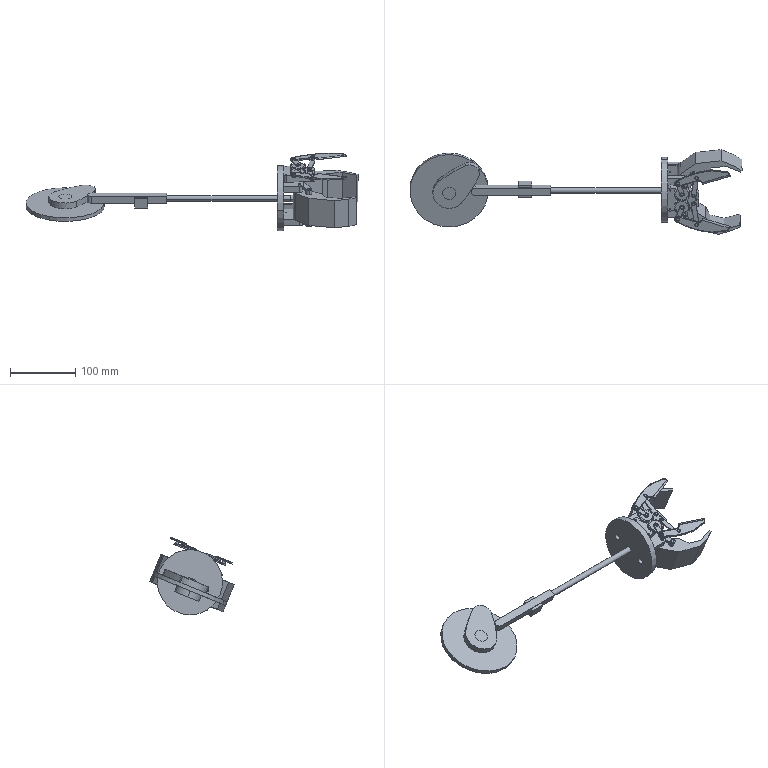Assembly | SolidWorks | mm | 30 component files | 31 solids | 649 faces | box 508.98 x 129.73 x 119.11 mm | volume 396416 mm3 | cylinder 341 | plane 286 | cone 16 | torus 4 | sphere 2 | commonest cylinder face diameters 4 x54 0.6 x54 5 x40 24 x40 5.6 x20 2.2 x14 8.636 x14 10 x12
Bill of materials:
2026.08.03FixedRail | 1 |  | Rectangular prismatic block with a rectangular slot running its full length, so its constant cross-section is a U-channel.
2026.08.03NewSchemeConnectingRod | 1 |  | Long straight bar with a square cross-section. One end is rounded. The other end face has a centered round blind hole whose bottom looks conical.
Cam | 1 |  | Flat plate of uniform thickness with a teardrop or cam-like outline. It has a single round through-hole near the center of the larger rounded end.
ConnectingRod | 2 |  | Flat straight link with an obround outline. It has two round through-holes, one at the center of each rounded end, and constant thickness.
ConnectingRod-B | 1 |  | Straight link with two through-holes. One end carries a taller cylindrical boss that sticks out from one face only, which gives an L-shaped side profile.
EccentricWheel | 1 |  | Thin circular disc with a small cylindrical pin or boss at its center. The pin appears to stick out from both faces.
FixedBushing | 1 |  | Plain thick ring with a rectangular cross-section: a cylindrical outer surface and a concentric cylindrical bore.
Holding Part | 1 |  | Thick plate with a trapezoidal outline and rounded corners. It has seven round through-holes: two small holes near the wide end, four larger holes in a roughly rectangular pattern, and one small hole near the narrow end.
Long Arm | 1 |  | Flat straight link with an obround outline and constant thickness. It has two round through-holes, one at the center of each rounded end.
MirrorConnectingRod-B | 1 |  | Straight link with two through-holes. A taller cylindrical boss at one end extends from one face, which gives an L-shaped side profile.
MirrorLong Arm | 1 |  | Flat straight link with an obround outline and constant thickness. It has two round through-holes, one at each rounded end.
Mirrorpin | 1 |  | Solid cylinder with a rectangular key or rib running lengthwise along one side. The key covers only part of the cylinder's length, starting at or near one end.
Mirrorpin2 | 3 |  | Plain solid right circular cylinder with flat ends.
MirrorShort Arm | 1 |  | Flat link plate (bar with rounded ends) with a through hole at each end; one hole has a small rectangular keyway notch.
MirrorSimple Gear | 1 |  | Flat spur-gear-like disc with straight-sided, roughly trapezoidal teeth and a central bore with keyway-type notches.
MirrorThe Claw | 1 |  | Thin flat blade-shaped plate with two small holes in a narrow shank and a wider tapering blade section with a bevelled edge.
Part1(1) | 1 |  | Circular flange disc with two parallel rectangular plate brackets sticking out from one face; the brackets and disc have several holes.
pin | 1 |  | Solid cylinder with a rectangular key-like rib running along the full length of its side.
pin2 | 3 |  | Plain solid right circular cylinder with flat ends.
RightJaw | 2 |  | Thick bracket or lever with a bent profile: one rounded end with a through hole, a small cylindrical pin sticking out of both faces, and an angled arm.
Short Arm | 1 |  | Flat link plate with rounded ends and two end holes; one hole has a small keyway notch.
Simple Gear | 1 |  | Flat spur-gear-like disc with straight-sided teeth and a central bore with keyway-type notches.
TelescopicRod | 1 |  | Long thin round rod ending in a short perpendicular cross-bar, forming a T, with a ball-shaped node where they meet.
The Claw | 1 |  | Thin flat blade-shaped plate with two holes in a narrow shank and a wider section with a bevelled long edge and an angled tip.
Mates:
1. concentric | Part1(1)-1 face at (323.621, 37.527, 8.706) dir (0, 0.3818, -0.9242) r 2.5 | RightJaw-1 face at (323.621, 20.343, 50.296) dir (0, 0.3818, -0.9242) r 2.5
2. coincident | Part1(1)-1 face at (328.621, 42.148, 10.615) dir (0, -0.3818, 0.9242) | RightJaw-2 face at (323.621, -13.306, -12.296) dir (0, 0.3818, -0.9242)
3. concentric | Part1(1)-1 face at (323.621, -13.306, -12.296) dir (0, 0.3818, -0.9242) r 2.5 | RightJaw-2 face at (323.621, -13.306, -12.296) dir (0, -0.3818, 0.9242) r 2.5
4. concentric | RightJaw-1 face at (338.214, 48.015, 4.383) dir (0, -0.3818, 0.9242) r 2.5 | ConnectingRod-1 face at (338.214, 46.488, 8.08) dir (0, -0.3818, 0.9242) r 2.5
5. coincident | RightJaw-1 face at (323.621, 37.527, 8.706) dir (0, 0.3818, -0.9242) | ConnectingRod-1 face at (338.214, 44.961, 11.777) dir (0, -0.3818, 0.9242)
6. concentric | RightJaw-2 face at (337.105, -19.3, -23.428) dir (0, -0.3818, 0.9242) r 2.5 | ConnectingRod-B-1 face at (337.105, -20.827, -19.731) dir (0, 0.3818, -0.9242) r 2.5
7. concentric | TelescopicRod-1 face at (321.124, -8.702, 46.952) dir (0, 0.3818, -0.9242) r 2.5 | ConnectingRod-1 face at (321.124, 13.063, -5.729) dir (0, -0.3818, 0.9242) r 2.5
8. concentric | TelescopicRod-1 face at (321.124, -8.702, 46.952) dir (0, 0.3818, -0.9242) r 2.5 | ConnectingRod-B-1 face at (321.124, 13.063, -5.729) dir (0, 0.3818, -0.9242) r 2.5
9. coincident | ConnectingRod-1 face at (338.214, 46.488, 8.08) dir (0, 0.3818, -0.9242) | ConnectingRod-B-1 face at (321.124, 13.063, -5.729) dir (0, -0.3818, 0.9242)
10. coincident | ConnectingRod-2 face at (338.214, 26.25, 57.064) dir (0, -0.3818, 0.9242) | MirrorConnectingRod-B-2 face at (321.124, -7.175, 43.255) dir (0, 0.3818, -0.9242)
11. parallel | 2026.08.03FixedRail-1 face at (90.094, 11.482, 13.811) dir (0, -0.3818, 0.9242) | 2026.08.03NewSchemeConnectingRod-2 face at (3.551, 0.6532, 24.308) dir (0, -0.3818, 0.9242)
12. parallel | Part1(1)-1 face at (328.621, -38.929, 36.627) dir (0, -0.3818, 0.9242) | FixedBushing-2 face at (-36.329, 4.513, 6.427) dir (0, -0.3818, 0.9242)
13. concentric | FixedBushing-2 face at (-36.329, 4.513, 6.427) dir (0, 0.3818, -0.9242) r 12.5 | EccentricWheel-2 face at (-36.329, 8.332, -2.815) dir (0, -0.3818, 0.9242) r 12.5
14. concentric | EccentricWheel-2 face at (-36.329, -1.596, 21.215) dir (0, 0.3818, -0.9242) r 10 | Cam-1 face at (-36.329, 2.222, 11.972) dir (0, -0.3818, 0.9242) r 10
15. coincident | EccentricWheel-2 face at (-36.329, 2.222, 11.972) dir (0, -0.3818, 0.9242) | Cam-1 face at (-93.023, 69.986, 39.969) dir (0, 0.3818, -0.9242)
16. coincident | FixedBushing-2 face at (-36.329, 4.513, 6.427) dir (0, -0.3818, 0.9242) | EccentricWheel-2 face at (-36.329, 4.513, 6.427) dir (0, 0.3818, -0.9242)
17. coincident | 2026.08.03NewSchemeConnectingRod-2 face at (3.551, 5.235, 13.217) dir (0, 0.3818, -0.9242) | EccentricWheel-2 face at (-36.329, 2.222, 11.972) dir (0, -0.3818, 0.9242)
18. cam | Cam-1 face at (-181.218, 104.23, 64.937) dir (0, 0.3818, -0.9242) r 209.672 | 2026.08.03NewSchemeConnectingRod-2 face at (3.551, 0.6532, 24.308) dir (0, 0.3818, -0.9242) r 6
19. coincident | 2026.08.03FixedRail-1 face at (90.094, 0.3913, 9.229) dir (0, 0.9242, 0.3818) | 2026.08.03NewSchemeConnectingRod-2 face at (3.551, -4.892, 22.017) dir (0, -0.9242, -0.3818)
20. concentric | Part1(1)-1 face at (302.621, -16.981, 34.875) dir (0, -0.3818, 0.9242) r 1.1 | Holding Part-1 face at (302.621, -25.381, 55.208) dir (0, 0.3818, -0.9242) r 1.1
21. coincident | Part1(1)-1 face at (302.621, 11.176, 46.508) dir (0, -0.3818, 0.9242) r 1.1 | Holding Part-1 edge at (302.621, 2.775, 66.841) dir (0, -0.3818, 0.9242) r 1.1
22. coincident | Part1(1)-1 face at (328.621, -38.929, 36.627) dir (0, -0.3818, 0.9242) | Holding Part-1 face at (342.621, 0.8389, 53.057) dir (0, 0.3818, -0.9242)
23. coincident | Holding Part-1 face at (320.621, -0.9517, 65.301) dir (0, 0.3818, -0.9242) r 2 | Simple Gear-1 edge at (320.621, -2.479, 68.998) dir (0, 0.3818, -0.9242) r 2
24. coincident | Holding Part-1 face at (342.621, -3.743, 64.148) dir (0, -0.3818, 0.9242) | Simple Gear-1 face at (320.621, -0.9517, 65.301) dir (0, 0.3818, -0.9242)
25. concentric | Short Arm-1 face at (320.621, -2.479, 68.998) dir (0, -0.3818, 0.9242) r 2 | Simple Gear-1 face at (320.621, -0.9517, 65.301) dir (0, -0.3818, 0.9242) r 2
26. coincident | Short Arm-1 face at (320.621, -2.479, 68.998) dir (0, 0.3818, -0.9242) | Simple Gear-1 face at (320.621, -2.479, 68.998) dir (0, -0.3818, 0.9242)
27. concentric | Short Arm-1 face at (314.445, 14.655, 76.077) dir (0, -0.3818, 0.9242) r 2 | The Claw-1 face at (314.445, 13.127, 79.774) dir (0, 0.3818, -0.9242) r 2
28. coincident | Short Arm-1 face at (320.621, -3.243, 70.847) dir (0, -0.3818, 0.9242) | The Claw-1 face at (315.971, 9.49, 76.108) dir (0, 0.3818, -0.9242)
29. concentric | Holding Part-1 face at (338.621, -4.649, 63.774) dir (0, 0.3818, -0.9242) r 2 | Long Arm-1 face at (338.621, -4.649, 63.774) dir (0, -0.3818, 0.9242) r 2
30. coincident | Holding Part-1 face at (342.621, -3.743, 64.148) dir (0, -0.3818, 0.9242) | Long Arm-1 face at (338.621, -4.649, 63.774) dir (0, 0.3818, -0.9242)
31. concentric | The Claw-1 face at (343.013, 21.592, 83.271) dir (0, 0.3818, -0.9242) r 2 | pin2-2 face at (343.013, 23.883, 77.726) dir (0, -0.3818, 0.9242) r 2
32. coincident | The Claw-1 face at (315.971, 8.727, 77.956) dir (0, -0.3818, 0.9242) | pin2-2 face at (343.013, 21.592, 83.271) dir (0, -0.3818, 0.9242)
33. concentric | Long Arm-1 face at (343.013, 24.647, 75.878) dir (0, -0.3818, 0.9242) r 2 | pin2-2 face at (343.013, 23.883, 77.726) dir (0, -0.3818, 0.9242) r 2
34. concentric | The Claw-1 face at (314.445, 13.127, 79.774) dir (0, 0.3818, -0.9242) r 2 | pin2-3 face at (314.445, 15.418, 74.229) dir (0, -0.3818, 0.9242) r 2
35. coincident | The Claw-1 face at (315.971, 8.727, 77.956) dir (0, -0.3818, 0.9242) | pin2-3 face at (314.445, 13.127, 79.774) dir (0, -0.3818, 0.9242)
36. concentric | pin-1 face at (320.621, -3.243, 70.847) dir (0, 0.3818, -0.9242) r 2 | Short Arm-1 face at (320.621, -2.479, 68.998) dir (0, -0.3818, 0.9242) r 2
37. coincident | pin-1 face at (321.095, -1.417, 66.841) dir (0.9487, 0.2921, 0.1207) | Short Arm-1 face at (321.095, -3.097, 70.907) dir (-0.9487, -0.2921, -0.1207)
38. coincident | pin-1 face at (320.621, -3.243, 70.847) dir (0, -0.3818, 0.9242) | Short Arm-1 face at (320.621, -3.243, 70.847) dir (0, -0.3818, 0.9242)
39. concentric | Long Arm-1 face at (338.621, -4.649, 63.774) dir (0, -0.3818, 0.9242) r 2 | pin2-4 face at (338.621, -3.121, 60.077) dir (0, -0.3818, 0.9242) r 2
40. coincident | Long Arm-1 face at (338.621, -5.412, 65.623) dir (0, -0.3818, 0.9242) | pin2-4 face at (338.621, -5.412, 65.623) dir (0, -0.3818, 0.9242)
41. distance | 2026.08.03NewSchemeConnectingRod-2 face at (119.194, 6.199, 26.599) dir (1, 0, 0) | TelescopicRod-1 face at (79.124, 2.944, 18.763) dir (-1, 0, 0)
42. concentric | TelescopicRod-1 face at (79.124, 2.944, 18.763) dir (1, 0, 0) r 5 | 2026.08.03NewSchemeConnectingRod-2 face at (119.194, 2.944, 18.763) dir (1, 0, 0) r 4.25
43. concentric | Mirrorpin-2 face at (320.621, -23.945, 62.293) dir (0, 0.3818, -0.9242) r 2 | MirrorSimple Gear-3 face at (320.621, -21.654, 56.748) dir (0, -0.3818, 0.9242) r 2
44. coincident | Holding Part-1 face at (342.621, -3.743, 64.148) dir (0, -0.3818, 0.9242) | MirrorSimple Gear-3 edge at (328.896, -26.601, 54.704) dir (0.997, -0.071, -0.02933)
45. gear | Simple Gear-1 face at (320.621, -0.9517, 65.301) dir (0, -0.3818, 0.9242) r 12 | MirrorSimple Gear-3 face at (320.621, -21.654, 56.748) dir (0, -0.3818, 0.9242) r 12
46. gear | MirrorShort Arm-2 face at (320.621, -23.182, 60.445) dir (0, -0.3818, 0.9242) r 2 | MirrorSimple Gear-3 face at (320.621, -21.654, 56.748) dir (0, -0.3818, 0.9242) r 2